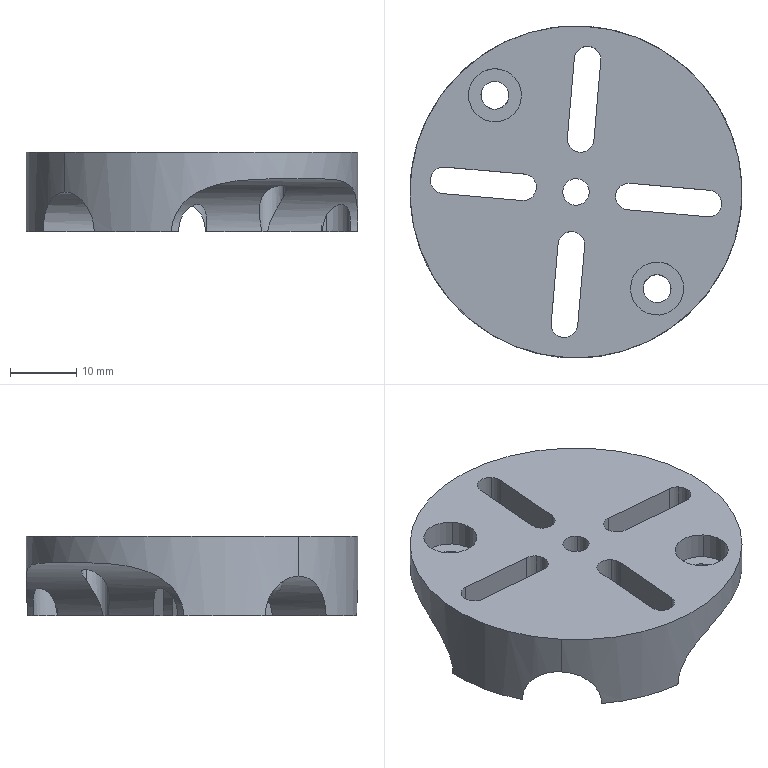Component | SolidWorks | LowerPartOfBracket-2 | 1 solid | 65 faces | box 50 x 50 x 12 mm | volume 12910 mm3 | cylinder 38 | plane 26 | sphere 1 | commonest cylinder face diameters 4 x16 8 x10 4.2 x4 12 x4 50 x2 16 x2
build123d program:
from build123d import *

# Parameters (mm, degrees)
SKETCH2_R                                           = 25
BOSS_EXTRUDE1_DEPTH                                 = 12
CUT_EXTRUDE1_DEPTH                                  = 38.336
CUT_EXTRUDE1_DEPTH_BACK                             = 38.336
SKETCH3_R                                           = 8
SKETCH3_R_2                                         = 6
CYLINDRICAL_COUNTERSUNK_HOLE_FOR_M6_HEX_D           = 4.2
CYLINDRICAL_COUNTERSUNK_HOLE_FOR_M6_HEX_DEPTH       = 38
CYLINDRICAL_COUNTERSUNK_HOLE_FOR_M6_HEX_CBORE_D     = 8
CYLINDRICAL_COUNTERSUNK_HOLE_FOR_M6_HEX_CBORE_DEPTH = 4
CYLINDRICAL_COUNTERSUNK_HOLE_FOR_M6_HEX_TIP         = 1.262
CUT_EXTRUDE2_DEPTH                                  = 38.336
CUT_EXTRUDE2_DEPTH_BACK                             = 38.336
CUT_EXTRUDE3_DEPTH                                  = 38.336
CUT_EXTRUDE3_DEPTH_BACK                             = 7
SKETCH10_R                                          = 2
BOSS_EXTRUDE2_DEPTH                                 = 7
DOME1_FACE_RADIUS                                   = 2
DOME1_HEIGHT                                        = 2
SKETCH11_R                                          = 2
CUT_EXTRUDE4_DEPTH                                  = 7


with BuildPart() as part:
    # Sketch2 → Boss-Extrude1 (new body)
    with BuildSketch(Plane(origin=(0, 0, 0), x_dir=(1, 0, 0), z_dir=(0, 1, 0))):
        with Locations(Location((0, 0, 0), (0, 0, 270))):
            Circle(SKETCH2_R)
    extrude(amount=BOSS_EXTRUDE1_DEPTH)

    # Sketch3 → Cut-Extrude1 (cut, two sides: drawn at the far end of the back side and taken through both)
    with BuildSketch(Plane.XY.offset(-CUT_EXTRUDE1_DEPTH_BACK)):
        with Locations((-25, 12)):
            Circle(SKETCH3_R)
        with Locations((25, 12)):
            Circle(SKETCH3_R)
        with Locations((0, 12)):
            Circle(SKETCH3_R_2)
    extrude(amount=CUT_EXTRUDE1_DEPTH + CUT_EXTRUDE1_DEPTH_BACK, mode=Mode.SUBTRACT)

    # Cylindrical Countersunk Hole for M6 Hex
    with Locations(Plane.XZ):
        with Locations((19, 0), (-19, 0)):
            CounterBoreHole(CYLINDRICAL_COUNTERSUNK_HOLE_FOR_M6_HEX_D / 2, CYLINDRICAL_COUNTERSUNK_HOLE_FOR_M6_HEX_CBORE_D / 2, CYLINDRICAL_COUNTERSUNK_HOLE_FOR_M6_HEX_CBORE_DEPTH, depth=CYLINDRICAL_COUNTERSUNK_HOLE_FOR_M6_HEX_DEPTH)
            with Locations((0, 0, -(CYLINDRICAL_COUNTERSUNK_HOLE_FOR_M6_HEX_DEPTH + CYLINDRICAL_COUNTERSUNK_HOLE_FOR_M6_HEX_TIP / 2))):  # 118° drill point
                Cone(0, CYLINDRICAL_COUNTERSUNK_HOLE_FOR_M6_HEX_D / 2, CYLINDRICAL_COUNTERSUNK_HOLE_FOR_M6_HEX_TIP, mode=Mode.SUBTRACT)

    # Sketch6 → Cut-Extrude2 (cut, two sides: drawn at the far end of the back side and taken through both)
    with BuildSketch(Plane.XZ.offset(-CUT_EXTRUDE2_DEPTH_BACK)):
        with BuildLine():
            Line((4.243, 7.071), (12.728, 15.556))
            ThreePointArc((12.728, 15.556), (15.556, 15.556), (15.556, 12.728))
            Line((15.556, 12.728), (7.071, 4.243))
            ThreePointArc((7.071, 4.243), (4.243, 4.243), (4.243, 7.071))
        make_face()
        with BuildLine():
            Line((7.071, -4.243), (15.556, -12.728))
            ThreePointArc((15.556, -12.728), (15.556, -15.556), (12.728, -15.556))
            Line((12.728, -15.556), (4.243, -7.071))
            ThreePointArc((4.243, -7.071), (4.243, -4.243), (7.071, -4.243))
        make_face()
        with BuildLine():
            Line((-4.243, -7.071), (-12.728, -15.556))
            ThreePointArc((-12.728, -15.556), (-15.556, -15.556), (-15.556, -12.728))
            Line((-15.556, -12.728), (-7.071, -4.243))
            ThreePointArc((-7.071, -4.243), (-4.243, -4.243), (-4.243, -7.071))
        make_face()
        with BuildLine():
            Line((-7.071, 4.243), (-15.556, 12.728))
            ThreePointArc((-15.556, 12.728), (-15.556, 15.556), (-12.728, 15.556))
            Line((-12.728, 15.556), (-4.243, 7.071))
            ThreePointArc((-4.243, 7.071), (-4.243, 4.243), (-7.071, 4.243))
        make_face()
    extrude(amount=CUT_EXTRUDE2_DEPTH + CUT_EXTRUDE2_DEPTH_BACK, mode=Mode.SUBTRACT)

    # Sketch9 → Cut-Extrude3 (cut, two sides: drawn at the far end of the back side and taken through both)
    with BuildSketch(Plane(origin=(0, 12, 0), x_dir=(1, 0, 0), z_dir=(0, 1, 0)).offset(-CUT_EXTRUDE3_DEPTH_BACK)):
        with BuildLine():
            Line((-11.314, 16.971), (16.971, -11.314))
            ThreePointArc((16.971, -11.314), (16.971, -16.971), (11.314, -16.971))
            Line((11.314, -16.971), (-16.971, 11.314))
            ThreePointArc((-16.971, 11.314), (-16.971, 16.971), (-11.314, 16.971))
        make_face()
        with BuildLine():
            Line((-16.971, -11.314), (11.314, 16.971))
            ThreePointArc((11.314, 16.971), (16.971, 16.971), (16.971, 11.314))
            Line((16.971, 11.314), (-11.314, -16.971))
            ThreePointArc((-11.314, -16.971), (-16.971, -16.971), (-16.971, -11.314))
        make_face()
    extrude(amount=CUT_EXTRUDE3_DEPTH + CUT_EXTRUDE3_DEPTH_BACK, mode=Mode.SUBTRACT)

    # Sketch10 → Boss-Extrude2 (add)
    with BuildSketch(Plane.XZ):
        with Locations(Location((0, 18, 0), (0, 0, 270))):
            Circle(SKETCH10_R)
    extrude(amount=-BOSS_EXTRUDE2_DEPTH)

    # Dome1: a dome of height H over a round flat face of radius A is a cap of a sphere of radius (A * A + H * H) / (2 * H)
    dome1_r = (DOME1_FACE_RADIUS * DOME1_FACE_RADIUS + DOME1_HEIGHT * DOME1_HEIGHT) / (2 * DOME1_HEIGHT)
    dome1_base = Plane((0, 7, 18), z_dir=(0, 1, 0))
    with Locations(dome1_base.offset(DOME1_HEIGHT - dome1_r)):
        dome1_ball = Sphere(dome1_r, mode=Mode.PRIVATE)
    add(split(dome1_ball, bisect_by=dome1_base, keep=Keep.TOP, mode=Mode.PRIVATE))

    # Sketch11 → Cut-Extrude4 (cut)
    with BuildSketch(Plane.XZ):
        with Locations(Location((0, 0, 0), (0, 0, 270))):
            Circle(SKETCH11_R)
    extrude(amount=-CUT_EXTRUDE4_DEPTH, mode=Mode.SUBTRACT)


solid = part.part

# Placed as in the assembly
solid = solid.moved(Location((-179.217, -162.42, 1039.6), (90, -49.999, -180)))